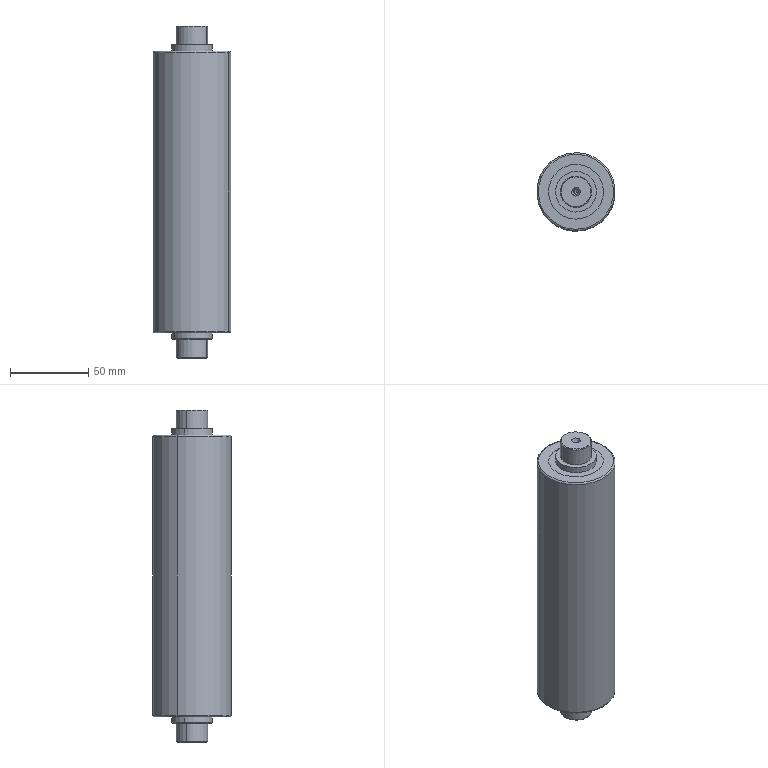Component | SolidWorks | 8TC-A15004-D0-06A-1 | 2 solids | 44 faces | box 50 x 50 x 212 mm | volume 365003 mm3 | cylinder 18 | cone 14 | plane 8 | torus 4 | commonest cylinder face diameters 3 x4 26 x4 20 x4 35 x4 50 x2 | material #45
build123d program:
from build123d import *

# Parameters (mm, degrees)
FILLET1_R              = 1
CHAMFER1_SIZE          = 0.5
SPLIT1_SURFACE_1_BACK  = 224.482
SPLIT1_SURFACE_1_DEPTH = 448.964
SPLIT1_SURFACE_2_BACK  = 224.482
SPLIT1_SURFACE_2_DEPTH = 448.964


with BuildPart() as part:
    # Sketch1 → Revolve1 (revolve)
    with BuildSketch(Plane(origin=(0, 0, 0), x_dir=(1, 0, 0), z_dir=(0, 1, 0)), mode=Mode.PRIVATE) as revolve1_sk:
        Polygon((0, 0), (0, 10), (12, 10), (12, 13), (16, 13), (16, 25), (196, 25), (196, 13), (200, 13), (200, 10), (212, 10), (212, 0), align=None)
    revolve(revolve1_sk.sketch.rotate(Axis((0, 0, 0), (1, 0, 0)), 180), axis=Axis((0, 0, 0), (1, 0, 0)))

    # Fillet1
    fillet1_edges = [part.edges().sort_by_distance(p)[0] for p in [
        (196, 0, -25),
        (16, 0, -25),
    ]]
    fillet(fillet1_edges, radius=FILLET1_R)

    # Chamfer1
    chamfer1_edges = [part.edges().sort_by_distance(p)[0] for p in [
        (12, 0, -13),
        (0, 0, -10),
        (212, 0, -10),
    ]]
    chamfer(chamfer1_edges, length=CHAMFER1_SIZE)


with BuildPart() as body_2:
    # Split1: the piece behind the surface
    add(part.part)
    # Split1 surface: a surface, the sketch's curves swept straight by 448.964 mm
    with BuildLine(Plane(origin=(196, 0, 0), x_dir=(0, 0, -1), z_dir=(1, 0, 0)).offset(-SPLIT1_SURFACE_1_BACK), mode=Mode.PRIVATE) as split1_surface_1_path:
        CenterArc((0, 0), 17.5, 0, 360)
    split1_surface_1 = Shell.extrude(split1_surface_1_path.wire(), (1 * SPLIT1_SURFACE_1_DEPTH, 0 * SPLIT1_SURFACE_1_DEPTH, 0 * SPLIT1_SURFACE_1_DEPTH))
    split(bisect_by=split1_surface_1, keep=Keep.BOTTOM)


with BuildPart() as part_1:
    add(part.part)

    # Split1: split by a surface, the side it looks to stays
    # Split1 surface: a surface, the sketch's curves swept straight by 448.964 mm
    with BuildLine(Plane(origin=(196, 0, 0), x_dir=(0, 0, -1), z_dir=(1, 0, 0)).offset(-SPLIT1_SURFACE_2_BACK), mode=Mode.PRIVATE) as split1_surface_2_path:
        CenterArc((0, 0), 17.5, 0, 360)
    split1_surface_2 = Shell.extrude(split1_surface_2_path.wire(), (1 * SPLIT1_SURFACE_2_DEPTH, 0 * SPLIT1_SURFACE_2_DEPTH, 0 * SPLIT1_SURFACE_2_DEPTH))
    split(bisect_by=split1_surface_2, keep=Keep.TOP)

    # Sketch3 → Cut-Revolve1 (revolve, cut)
    with BuildSketch(Plane.XY, mode=Mode.PRIVATE) as cut_revolve1_sk:
        Polygon((0, 0), (0, 2.743), (3, 1.5), (5.099, 1.5), (6, 0), align=None)
        Polygon((206, 0), (212, 0), (212, 2.743), (209, 1.5), (206.901, 1.5), align=None)
    revolve(cut_revolve1_sk.sketch.rotate(Axis((0, 0, 0), (1, 0, 0)), 90), axis=Axis((0, 0, 0), (1, 0, 0)), mode=Mode.SUBTRACT)


solid = Compound([body_2.part, part_1.part])

# Placed as in the assembly
solid = solid.moved(Location((-7.5, 286.5, -106), (0, -90, 0)))